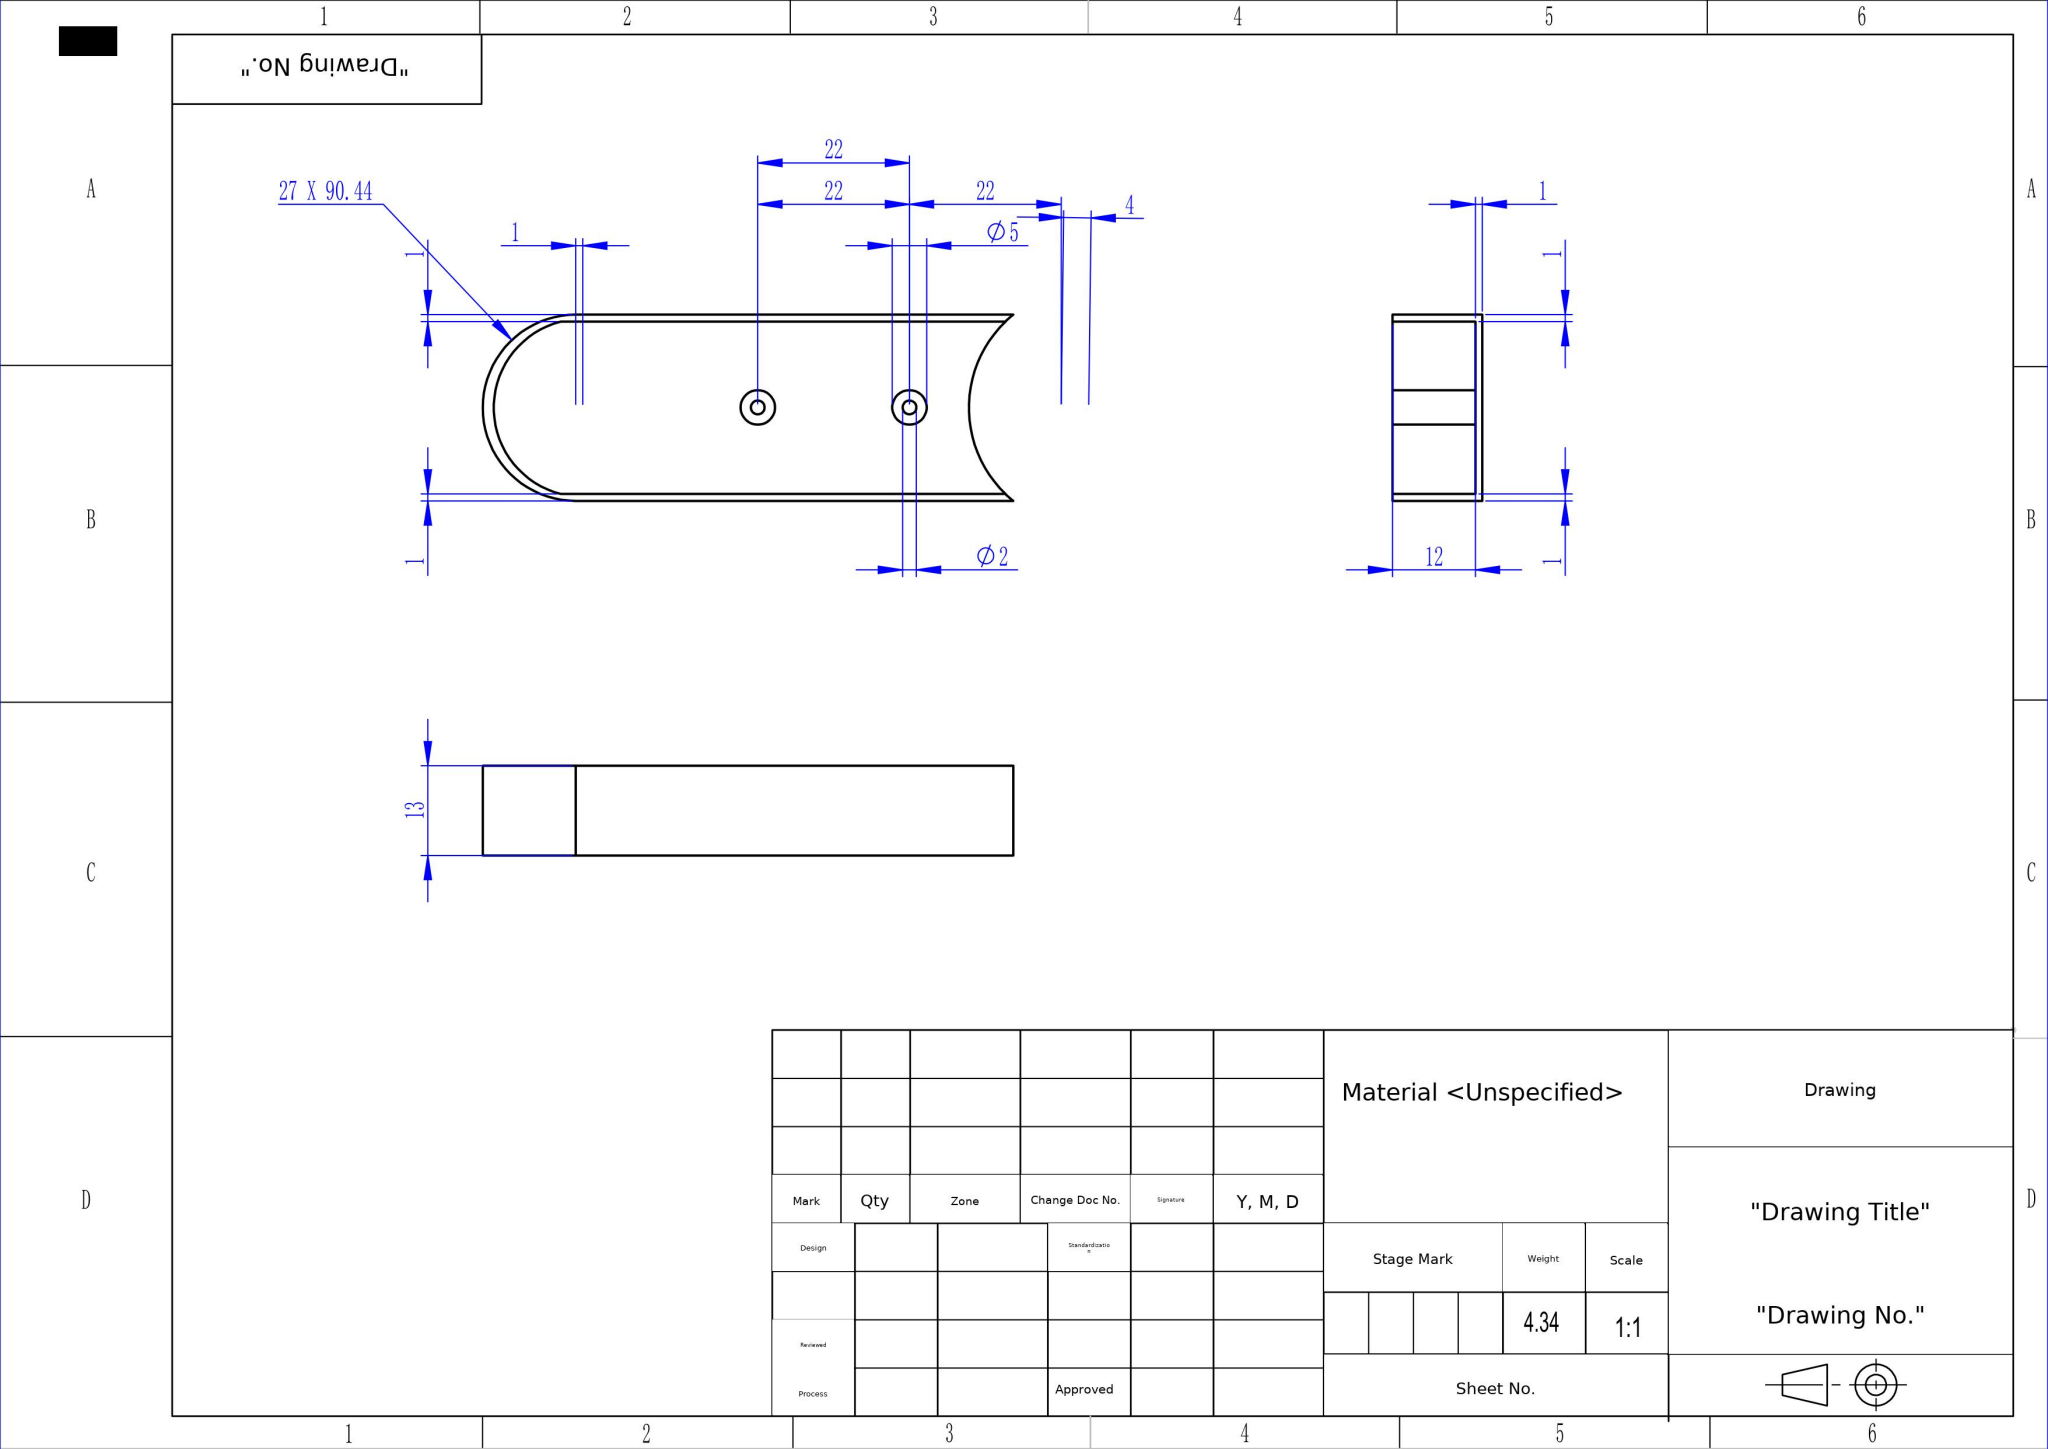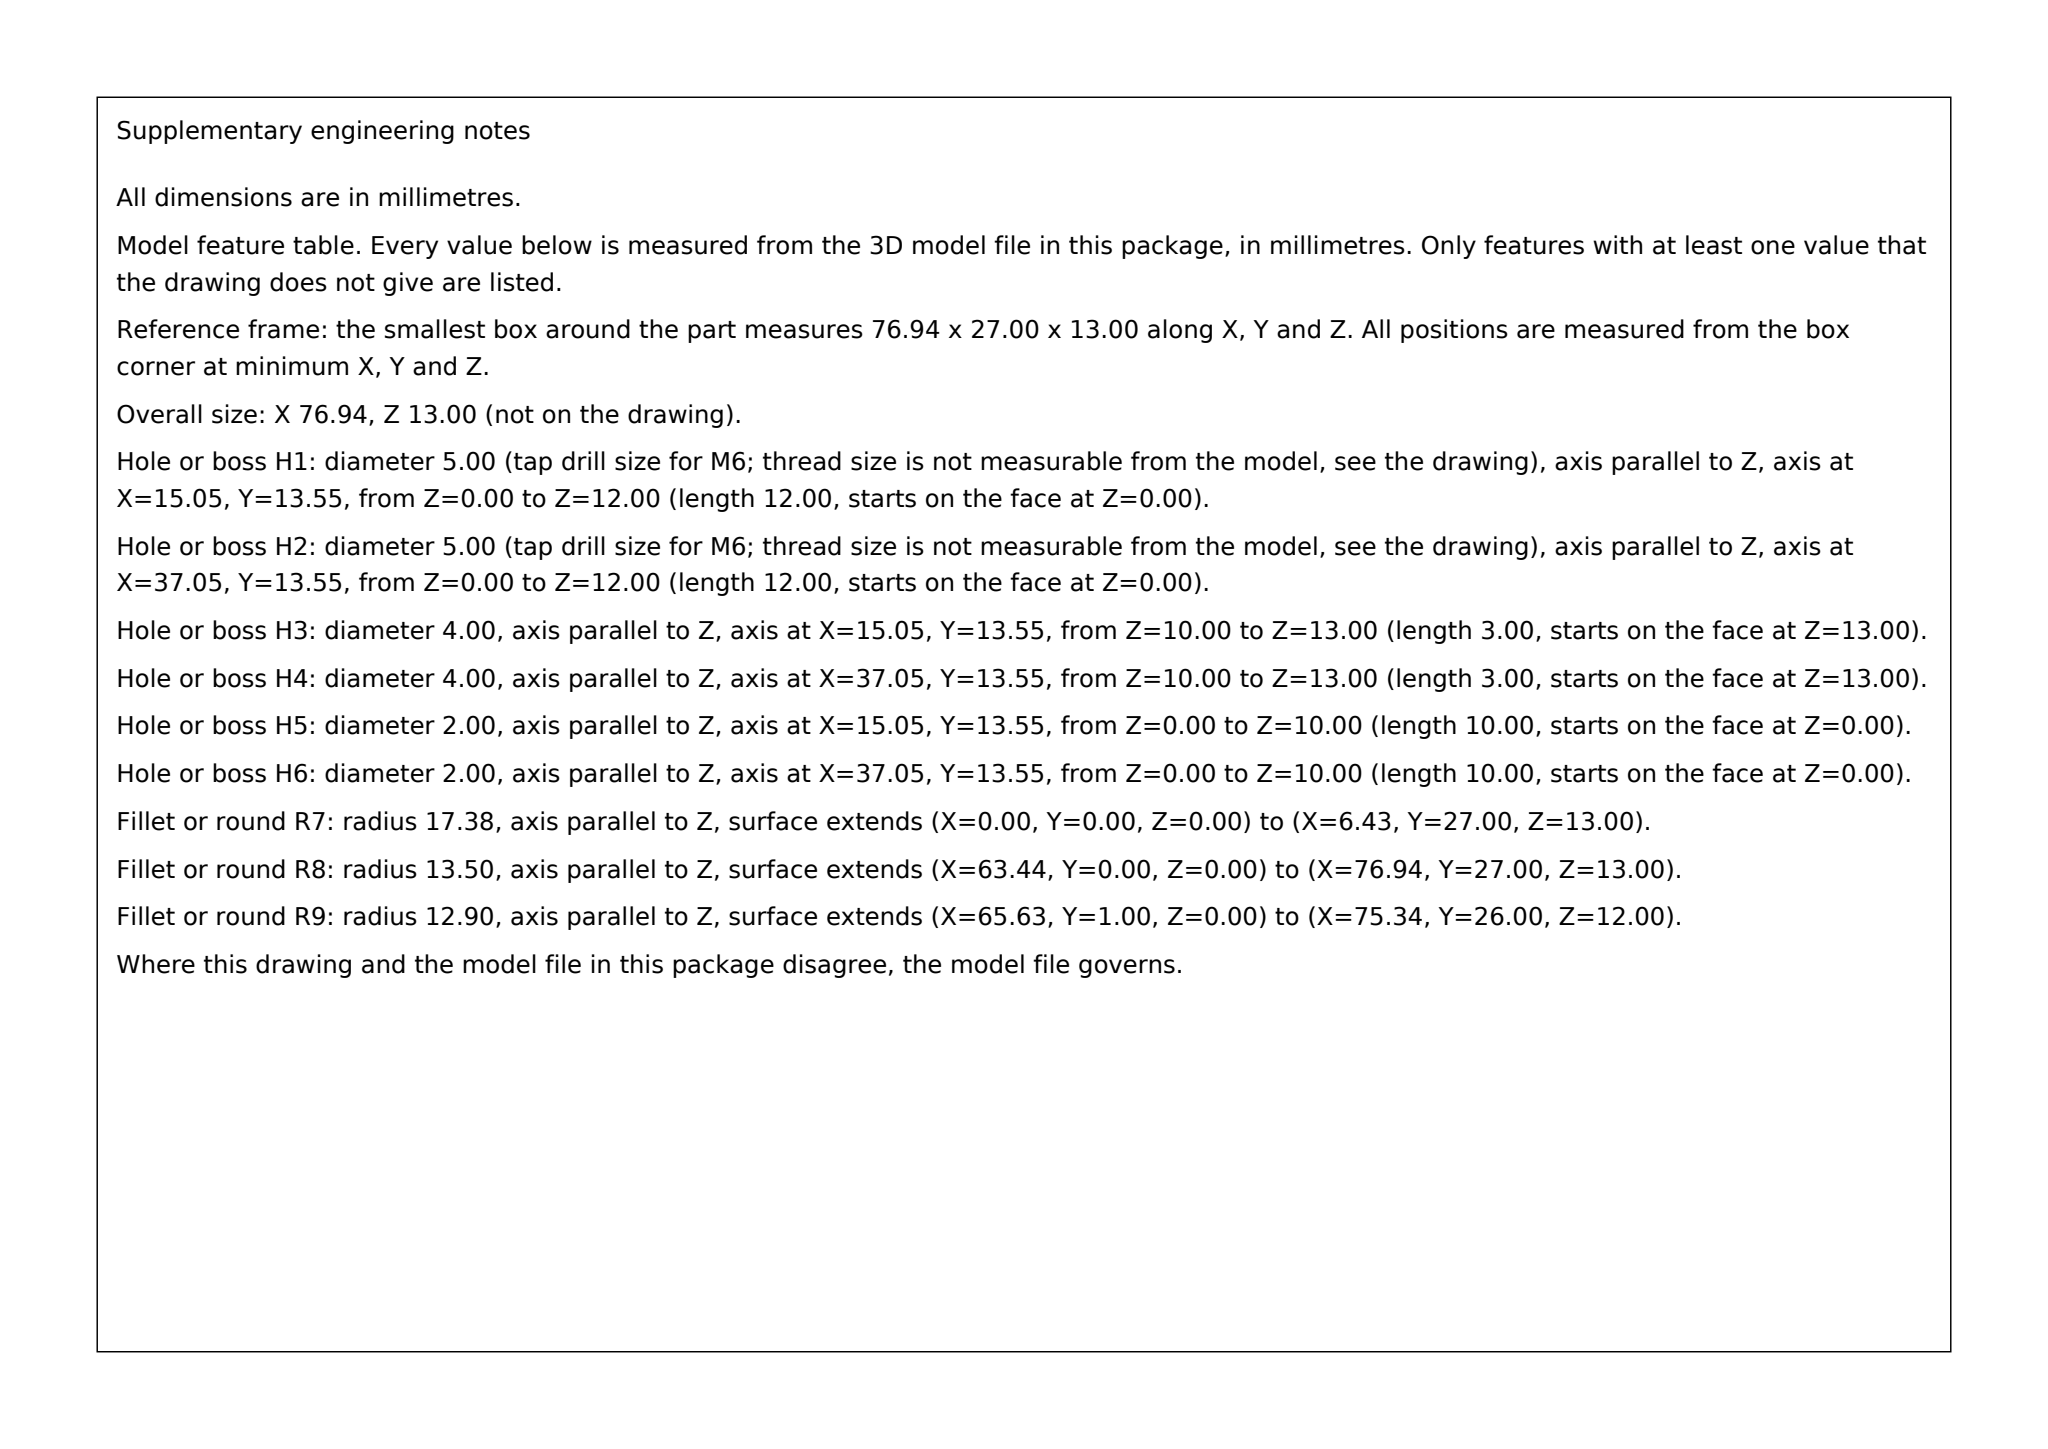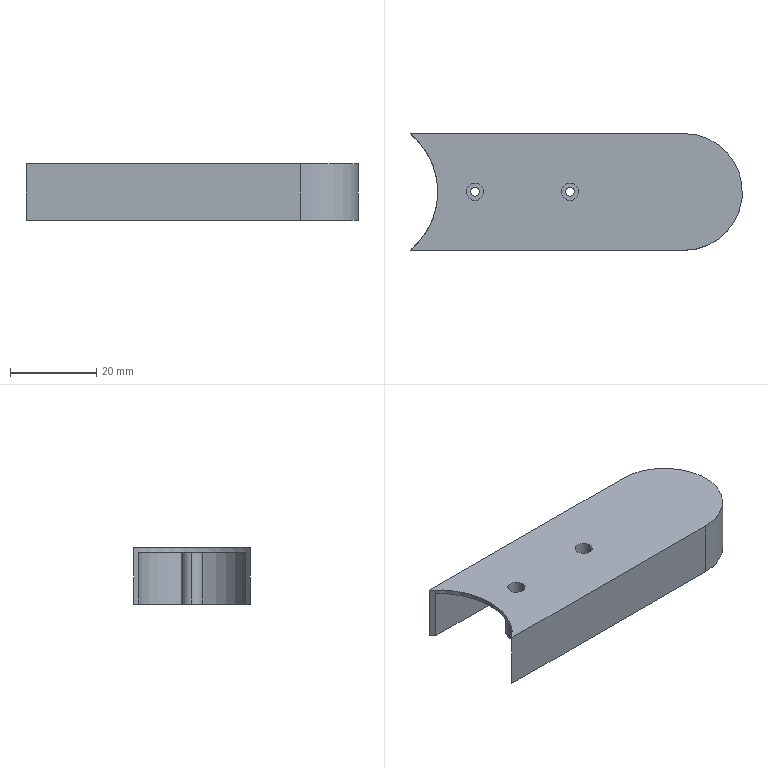Part | SolidWorks | mm | 1 solid | 26 faces | box 76.94 x 27 x 13 mm | volume 4339 mm3 | cylinder 15 | plane 11 | commonest cylinder face diameters 4 x4 5 x4 2 x4 34.768 x1 27 x1 25.801 x1
STEP:
#1=CARTESIAN_POINT('',(-54.,-0.,10.));
#2=VERTEX_POINT('',#1);
#3=CARTESIAN_POINT('',(-50.,-0.,10.));
#4=VERTEX_POINT('',#3);
#5=CARTESIAN_POINT('',(-52.,-0.,10.));
#6=DIRECTION('',(0.,0.,1.));
#7=DIRECTION('',(1.,0.,0.));
#8=AXIS2_PLACEMENT_3D('',#5,#6,#7);
#9=CIRCLE('',#8,2.);
#10=EDGE_CURVE('',#2,#4,#9,.T.);
#11=ORIENTED_EDGE('',*,*,#10,.F.);
#12=CARTESIAN_POINT('',(-54.,-0.,13.));
#13=VERTEX_POINT('',#12);
#14=CARTESIAN_POINT('',(-54.,-0.,10.));
#15=DIRECTION('',(0.,0.,1.));
#16=VECTOR('',#15,1000.);
#17=LINE('',#14,#16);
#18=EDGE_CURVE('',#2,#13,#17,.T.);
#19=ORIENTED_EDGE('',*,*,#18,.T.);
#20=CARTESIAN_POINT('',(-50.,-0.,13.));
#21=VERTEX_POINT('',#20);
#22=CARTESIAN_POINT('',(-52.,-0.,13.));
#23=DIRECTION('',(0.,0.,1.));
#24=DIRECTION('',(1.,0.,0.));
#25=AXIS2_PLACEMENT_3D('',#22,#23,#24);
#26=CIRCLE('',#25,2.);
#27=EDGE_CURVE('',#13,#21,#26,.T.);
#28=ORIENTED_EDGE('',*,*,#27,.T.);
#29=CARTESIAN_POINT('',(-50.,-0.,10.));
#30=DIRECTION('',(0.,0.,1.));
#31=VECTOR('',#30,1000.);
#32=LINE('',#29,#31);
#33=EDGE_CURVE('',#4,#21,#32,.T.);
#34=ORIENTED_EDGE('',*,*,#33,.F.);
#35=EDGE_LOOP('',(#11,#19,#28,#34));
#36=FACE_OUTER_BOUND('',#35,.T.);
#37=CARTESIAN_POINT('',(-52.,-0.,10.));
#38=DIRECTION('',(0.,0.,1.));
#39=DIRECTION('',(1.,0.,0.));
#40=AXIS2_PLACEMENT_3D('',#37,#38,#39);
#41=CYLINDRICAL_SURFACE('',#40,2.);
#42=ADVANCED_FACE('',(#36),#41,.F.);
#43=CARTESIAN_POINT('',(-76.,0.,10.));
#44=VERTEX_POINT('',#43);
#45=CARTESIAN_POINT('',(-72.,0.,10.));
#46=VERTEX_POINT('',#45);
#47=CARTESIAN_POINT('',(-74.,0.,10.));
#48=DIRECTION('',(0.,0.,1.));
#49=DIRECTION('',(1.,0.,0.));
#50=AXIS2_PLACEMENT_3D('',#47,#48,#49);
#51=CIRCLE('',#50,2.);
#52=EDGE_CURVE('',#44,#46,#51,.T.);
#53=ORIENTED_EDGE('',*,*,#52,.F.);
#54=CARTESIAN_POINT('',(-76.,0.,13.));
#55=VERTEX_POINT('',#54);
#56=CARTESIAN_POINT('',(-76.,0.,10.));
#57=DIRECTION('',(0.,0.,1.));
#58=VECTOR('',#57,1000.);
#59=LINE('',#56,#58);
#60=EDGE_CURVE('',#44,#55,#59,.T.);
#61=ORIENTED_EDGE('',*,*,#60,.T.);
#62=CARTESIAN_POINT('',(-72.,0.,13.));
#63=VERTEX_POINT('',#62);
#64=CARTESIAN_POINT('',(-74.,0.,13.));
#65=DIRECTION('',(0.,0.,1.));
#66=DIRECTION('',(1.,0.,0.));
#67=AXIS2_PLACEMENT_3D('',#64,#65,#66);
#68=CIRCLE('',#67,2.);
#69=EDGE_CURVE('',#55,#63,#68,.T.);
#70=ORIENTED_EDGE('',*,*,#69,.T.);
#71=CARTESIAN_POINT('',(-72.,0.,10.));
#72=DIRECTION('',(0.,0.,1.));
#73=VECTOR('',#72,1000.);
#74=LINE('',#71,#73);
#75=EDGE_CURVE('',#46,#63,#74,.T.);
#76=ORIENTED_EDGE('',*,*,#75,.F.);
#77=EDGE_LOOP('',(#53,#61,#70,#76));
#78=FACE_OUTER_BOUND('',#77,.T.);
#79=CARTESIAN_POINT('',(-74.,0.,10.));
#80=DIRECTION('',(0.,0.,1.));
#81=DIRECTION('',(1.,0.,0.));
#82=AXIS2_PLACEMENT_3D('',#79,#80,#81);
#83=CYLINDRICAL_SURFACE('',#82,2.);
#84=ADVANCED_FACE('',(#78),#83,.F.);
#85=CARTESIAN_POINT('',(-54.5,-0.,-0.));
#86=VERTEX_POINT('',#85);
#87=CARTESIAN_POINT('',(-49.5,-0.,-0.));
#88=VERTEX_POINT('',#87);
#89=CARTESIAN_POINT('',(-52.,-0.,-0.));
#90=DIRECTION('',(0.,0.,-1.));
#91=DIRECTION('',(0.,1.,0.));
#92=AXIS2_PLACEMENT_3D('',#89,#90,#91);
#93=CIRCLE('',#92,2.5);
#94=EDGE_CURVE('',#86,#88,#93,.T.);
#95=ORIENTED_EDGE('',*,*,#94,.F.);
#96=CARTESIAN_POINT('',(-54.5,-0.,12.));
#97=VERTEX_POINT('',#96);
#98=CARTESIAN_POINT('',(-54.5,-0.,-7.071));
#99=DIRECTION('',(0.,0.,1.));
#100=VECTOR('',#99,1000.);
#101=LINE('',#98,#100);
#102=EDGE_CURVE('',#86,#97,#101,.T.);
#103=ORIENTED_EDGE('',*,*,#102,.T.);
#104=CARTESIAN_POINT('',(-49.5,-0.,12.));
#105=VERTEX_POINT('',#104);
#106=CARTESIAN_POINT('',(-52.,-0.,12.));
#107=DIRECTION('',(0.,0.,-1.));
#108=DIRECTION('',(-1.,0.,0.));
#109=AXIS2_PLACEMENT_3D('',#106,#107,#108);
#110=CIRCLE('',#109,2.5);
#111=EDGE_CURVE('',#97,#105,#110,.T.);
#112=ORIENTED_EDGE('',*,*,#111,.T.);
#113=CARTESIAN_POINT('',(-49.5,-0.,-7.071));
#114=DIRECTION('',(0.,0.,1.));
#115=VECTOR('',#114,1000.);
#116=LINE('',#113,#115);
#117=EDGE_CURVE('',#88,#105,#116,.T.);
#118=ORIENTED_EDGE('',*,*,#117,.F.);
#119=EDGE_LOOP('',(#95,#103,#112,#118));
#120=FACE_OUTER_BOUND('',#119,.T.);
#121=CARTESIAN_POINT('',(-52.,-0.,-7.071));
#122=DIRECTION('',(0.,0.,1.));
#123=DIRECTION('',(1.,0.,0.));
#124=AXIS2_PLACEMENT_3D('',#121,#122,#123);
#125=CYLINDRICAL_SURFACE('',#124,2.5);
#126=ADVANCED_FACE('',(#120),#125,.T.);
#127=CARTESIAN_POINT('',(-76.5,0.,-0.));
#128=VERTEX_POINT('',#127);
#129=CARTESIAN_POINT('',(-71.5,0.,-0.));
#130=VERTEX_POINT('',#129);
#131=CARTESIAN_POINT('',(-74.,0.,-0.));
#132=DIRECTION('',(0.,0.,-1.));
#133=DIRECTION('',(0.,1.,0.));
#134=AXIS2_PLACEMENT_3D('',#131,#132,#133);
#135=CIRCLE('',#134,2.5);
#136=EDGE_CURVE('',#128,#130,#135,.T.);
#137=ORIENTED_EDGE('',*,*,#136,.F.);
#138=CARTESIAN_POINT('',(-76.5,0.,12.));
#139=VERTEX_POINT('',#138);
#140=CARTESIAN_POINT('',(-76.5,0.,-7.071));
#141=DIRECTION('',(0.,0.,1.));
#142=VECTOR('',#141,1000.);
#143=LINE('',#140,#142);
#144=EDGE_CURVE('',#128,#139,#143,.T.);
#145=ORIENTED_EDGE('',*,*,#144,.T.);
#146=CARTESIAN_POINT('',(-71.5,0.,12.));
#147=VERTEX_POINT('',#146);
#148=CARTESIAN_POINT('',(-74.,0.,12.));
#149=DIRECTION('',(0.,0.,-1.));
#150=DIRECTION('',(-1.,0.,0.));
#151=AXIS2_PLACEMENT_3D('',#148,#149,#150);
#152=CIRCLE('',#151,2.5);
#153=EDGE_CURVE('',#139,#147,#152,.T.);
#154=ORIENTED_EDGE('',*,*,#153,.T.);
#155=CARTESIAN_POINT('',(-71.5,0.,-7.071));
#156=DIRECTION('',(0.,0.,1.));
#157=VECTOR('',#156,1000.);
#158=LINE('',#155,#157);
#159=EDGE_CURVE('',#130,#147,#158,.T.);
#160=ORIENTED_EDGE('',*,*,#159,.F.);
#161=EDGE_LOOP('',(#137,#145,#154,#160));
#162=FACE_OUTER_BOUND('',#161,.T.);
#163=CARTESIAN_POINT('',(-74.,0.,-7.071));
#164=DIRECTION('',(0.,0.,1.));
#165=DIRECTION('',(1.,0.,0.));
#166=AXIS2_PLACEMENT_3D('',#163,#164,#165);
#167=CYLINDRICAL_SURFACE('',#166,2.5);
#168=ADVANCED_FACE('',(#162),#167,.T.);
#169=CARTESIAN_POINT('',(-75.,0.,-0.));
#170=VERTEX_POINT('',#169);
#171=CARTESIAN_POINT('',(-73.,0.,-0.));
#172=VERTEX_POINT('',#171);
#173=CARTESIAN_POINT('',(-74.,0.,-0.));
#174=DIRECTION('',(0.,0.,1.));
#175=DIRECTION('',(1.,0.,0.));
#176=AXIS2_PLACEMENT_3D('',#173,#174,#175);
#177=CIRCLE('',#176,1.);
#178=EDGE_CURVE('',#170,#172,#177,.T.);
#179=ORIENTED_EDGE('',*,*,#178,.F.);
#180=CARTESIAN_POINT('',(-75.,0.,10.));
#181=VERTEX_POINT('',#180);
#182=CARTESIAN_POINT('',(-75.,0.,-0.));
#183=DIRECTION('',(0.,0.,1.));
#184=VECTOR('',#183,1000.);
#185=LINE('',#182,#184);
#186=EDGE_CURVE('',#170,#181,#185,.T.);
#187=ORIENTED_EDGE('',*,*,#186,.T.);
#188=CARTESIAN_POINT('',(-73.,0.,10.));
#189=VERTEX_POINT('',#188);
#190=CARTESIAN_POINT('',(-74.,0.,10.));
#191=DIRECTION('',(0.,0.,-1.));
#192=DIRECTION('',(1.,0.,0.));
#193=AXIS2_PLACEMENT_3D('',#190,#191,#192);
#194=CIRCLE('',#193,1.);
#195=EDGE_CURVE('',#189,#181,#194,.T.);
#196=ORIENTED_EDGE('',*,*,#195,.F.);
#197=CARTESIAN_POINT('',(-73.,0.,-0.));
#198=DIRECTION('',(0.,0.,1.));
#199=VECTOR('',#198,1000.);
#200=LINE('',#197,#199);
#201=EDGE_CURVE('',#172,#189,#200,.T.);
#202=ORIENTED_EDGE('',*,*,#201,.F.);
#203=EDGE_LOOP('',(#179,#187,#196,#202));
#204=FACE_OUTER_BOUND('',#203,.T.);
#205=CARTESIAN_POINT('',(-74.,0.,-0.));
#206=DIRECTION('',(0.,0.,1.));
#207=DIRECTION('',(1.,0.,0.));
#208=AXIS2_PLACEMENT_3D('',#205,#206,#207);
#209=CYLINDRICAL_SURFACE('',#208,1.);
#210=ADVANCED_FACE('',(#204),#209,.F.);
#211=CARTESIAN_POINT('',(-53.,-0.,-0.));
#212=VERTEX_POINT('',#211);
#213=CARTESIAN_POINT('',(-51.,-0.,-0.));
#214=VERTEX_POINT('',#213);
#215=CARTESIAN_POINT('',(-52.,-0.,-0.));
#216=DIRECTION('',(0.,0.,1.));
#217=DIRECTION('',(1.,0.,0.));
#218=AXIS2_PLACEMENT_3D('',#215,#216,#217);
#219=CIRCLE('',#218,1.);
#220=EDGE_CURVE('',#212,#214,#219,.T.);
#221=ORIENTED_EDGE('',*,*,#220,.F.);
#222=CARTESIAN_POINT('',(-53.,-0.,10.));
#223=VERTEX_POINT('',#222);
#224=CARTESIAN_POINT('',(-53.,-0.,-0.));
#225=DIRECTION('',(0.,0.,1.));
#226=VECTOR('',#225,1000.);
#227=LINE('',#224,#226);
#228=EDGE_CURVE('',#212,#223,#227,.T.);
#229=ORIENTED_EDGE('',*,*,#228,.T.);
#230=CARTESIAN_POINT('',(-51.,-0.,10.));
#231=VERTEX_POINT('',#230);
#232=CARTESIAN_POINT('',(-52.,-0.,10.));
#233=DIRECTION('',(0.,0.,-1.));
#234=DIRECTION('',(1.,0.,0.));
#235=AXIS2_PLACEMENT_3D('',#232,#233,#234);
#236=CIRCLE('',#235,1.);
#237=EDGE_CURVE('',#231,#223,#236,.T.);
#238=ORIENTED_EDGE('',*,*,#237,.F.);
#239=CARTESIAN_POINT('',(-51.,-0.,-0.));
#240=DIRECTION('',(0.,0.,1.));
#241=VECTOR('',#240,1000.);
#242=LINE('',#239,#241);
#243=EDGE_CURVE('',#214,#231,#242,.T.);
#244=ORIENTED_EDGE('',*,*,#243,.F.);
#245=EDGE_LOOP('',(#221,#229,#238,#244));
#246=FACE_OUTER_BOUND('',#245,.T.);
#247=CARTESIAN_POINT('',(-52.,-0.,-0.));
#248=DIRECTION('',(0.,0.,1.));
#249=DIRECTION('',(1.,0.,0.));
#250=AXIS2_PLACEMENT_3D('',#247,#248,#249);
#251=CYLINDRICAL_SURFACE('',#250,1.);
#252=ADVANCED_FACE('',(#246),#251,.F.);
#253=ORIENTED_EDGE('',*,*,#228,.F.);
#254=CARTESIAN_POINT('',(-52.,-0.,-0.));
#255=DIRECTION('',(0.,0.,1.));
#256=DIRECTION('',(1.,0.,0.));
#257=AXIS2_PLACEMENT_3D('',#254,#255,#256);
#258=CIRCLE('',#257,1.);
#259=EDGE_CURVE('',#214,#212,#258,.T.);
#260=ORIENTED_EDGE('',*,*,#259,.F.);
#261=ORIENTED_EDGE('',*,*,#243,.T.);
#262=CARTESIAN_POINT('',(-52.,-0.,10.));
#263=DIRECTION('',(0.,0.,-1.));
#264=DIRECTION('',(1.,0.,0.));
#265=AXIS2_PLACEMENT_3D('',#262,#263,#264);
#266=CIRCLE('',#265,1.);
#267=EDGE_CURVE('',#223,#231,#266,.T.);
#268=ORIENTED_EDGE('',*,*,#267,.F.);
#269=EDGE_LOOP('',(#253,#260,#261,#268));
#270=FACE_OUTER_BOUND('',#269,.T.);
#271=CARTESIAN_POINT('',(-52.,-0.,-0.));
#272=DIRECTION('',(0.,0.,1.));
#273=DIRECTION('',(1.,0.,0.));
#274=AXIS2_PLACEMENT_3D('',#271,#272,#273);
#275=CYLINDRICAL_SURFACE('',#274,1.);
#276=ADVANCED_FACE('',(#270),#275,.F.);
#277=ORIENTED_EDGE('',*,*,#186,.F.);
#278=CARTESIAN_POINT('',(-74.,0.,-0.));
#279=DIRECTION('',(0.,0.,1.));
#280=DIRECTION('',(1.,0.,0.));
#281=AXIS2_PLACEMENT_3D('',#278,#279,#280);
#282=CIRCLE('',#281,1.);
#283=EDGE_CURVE('',#172,#170,#282,.T.);
#284=ORIENTED_EDGE('',*,*,#283,.F.);
#285=ORIENTED_EDGE('',*,*,#201,.T.);
#286=CARTESIAN_POINT('',(-74.,0.,10.));
#287=DIRECTION('',(0.,0.,-1.));
#288=DIRECTION('',(1.,0.,0.));
#289=AXIS2_PLACEMENT_3D('',#286,#287,#288);
#290=CIRCLE('',#289,1.);
#291=EDGE_CURVE('',#181,#189,#290,.T.);
#292=ORIENTED_EDGE('',*,*,#291,.F.);
#293=EDGE_LOOP('',(#277,#284,#285,#292));
#294=FACE_OUTER_BOUND('',#293,.T.);
#295=CARTESIAN_POINT('',(-74.,0.,-0.));
#296=DIRECTION('',(0.,0.,1.));
#297=DIRECTION('',(1.,0.,0.));
#298=AXIS2_PLACEMENT_3D('',#295,#296,#297);
#299=CYLINDRICAL_SURFACE('',#298,1.);
#300=ADVANCED_FACE('',(#294),#299,.F.);
#301=CARTESIAN_POINT('',(-89.048,13.45,0.));
#302=VERTEX_POINT('',#301);
#303=CARTESIAN_POINT('',(-87.919,12.45,0.));
#304=VERTEX_POINT('',#303);
#305=CARTESIAN_POINT('',(-100.,-0.05,0.));
#306=DIRECTION('',(0.,0.,-1.));
#307=DIRECTION('',(1.,-0.,0.));
#308=AXIS2_PLACEMENT_3D('',#305,#306,#307);
#309=CIRCLE('',#308,17.384);
#310=EDGE_CURVE('',#302,#304,#309,.T.);
#311=ORIENTED_EDGE('',*,*,#310,.T.);
#312=CARTESIAN_POINT('',(-87.919,12.45,12.));
#313=VERTEX_POINT('',#312);
#314=CARTESIAN_POINT('',(-87.919,12.45,12.));
#315=DIRECTION('',(0.,0.,-1.));
#316=VECTOR('',#315,1000.);
#317=LINE('',#314,#316);
#318=EDGE_CURVE('',#313,#304,#317,.T.);
#319=ORIENTED_EDGE('',*,*,#318,.F.);
#320=CARTESIAN_POINT('',(-87.919,-12.55,12.));
#321=VERTEX_POINT('',#320);
#322=CARTESIAN_POINT('',(-100.,-0.05,12.));
#323=DIRECTION('',(0.,0.,1.));
#324=DIRECTION('',(-1.,0.,0.));
#325=AXIS2_PLACEMENT_3D('',#322,#323,#324);
#326=CIRCLE('',#325,17.384);
#327=EDGE_CURVE('',#321,#313,#326,.T.);
#328=ORIENTED_EDGE('',*,*,#327,.F.);
#329=CARTESIAN_POINT('',(-87.919,-12.55,0.));
#330=VERTEX_POINT('',#329);
#331=CARTESIAN_POINT('',(-87.919,-12.55,12.));
#332=DIRECTION('',(0.,0.,-1.));
#333=VECTOR('',#332,1000.);
#334=LINE('',#331,#333);
#335=EDGE_CURVE('',#321,#330,#334,.T.);
#336=ORIENTED_EDGE('',*,*,#335,.T.);
#337=CARTESIAN_POINT('',(-89.048,-13.55,0.));
#338=VERTEX_POINT('',#337);
#339=CARTESIAN_POINT('',(-100.,-0.05,0.));
#340=DIRECTION('',(0.,0.,-1.));
#341=DIRECTION('',(1.,0.,0.));
#342=AXIS2_PLACEMENT_3D('',#339,#340,#341);
#343=CIRCLE('',#342,17.384);
#344=EDGE_CURVE('',#330,#338,#343,.T.);
#345=ORIENTED_EDGE('',*,*,#344,.T.);
#346=CARTESIAN_POINT('',(-89.048,-13.55,13.));
#347=VERTEX_POINT('',#346);
#348=CARTESIAN_POINT('',(-89.048,-13.55,13.));
#349=DIRECTION('',(0.,0.,-1.));
#350=VECTOR('',#349,1000.);
#351=LINE('',#348,#350);
#352=EDGE_CURVE('',#347,#338,#351,.T.);
#353=ORIENTED_EDGE('',*,*,#352,.F.);
#354=CARTESIAN_POINT('',(-89.048,13.45,13.));
#355=VERTEX_POINT('',#354);
#356=CARTESIAN_POINT('',(-100.,-0.05,13.));
#357=DIRECTION('',(0.,0.,-1.));
#358=DIRECTION('',(1.,0.,0.));
#359=AXIS2_PLACEMENT_3D('',#356,#357,#358);
#360=CIRCLE('',#359,17.384);
#361=EDGE_CURVE('',#355,#347,#360,.T.);
#362=ORIENTED_EDGE('',*,*,#361,.F.);
#363=CARTESIAN_POINT('',(-89.048,13.45,13.));
#364=DIRECTION('',(0.,0.,-1.));
#365=VECTOR('',#364,1000.);
#366=LINE('',#363,#365);
#367=EDGE_CURVE('',#355,#302,#366,.T.);
#368=ORIENTED_EDGE('',*,*,#367,.T.);
#369=EDGE_LOOP('',(#311,#319,#328,#336,#345,#353,#362,#368));
#370=FACE_OUTER_BOUND('',#369,.T.);
#371=CARTESIAN_POINT('',(-100.,-0.05,13.));
#372=DIRECTION('',(0.,0.,-1.));
#373=DIRECTION('',(-1.,0.,0.));
#374=AXIS2_PLACEMENT_3D('',#371,#372,#373);
#375=CYLINDRICAL_SURFACE('',#374,17.384);
#376=ADVANCED_FACE('',(#370),#375,.F.);
#377=CARTESIAN_POINT('',(-25.611,-13.55,0.));
#378=VERTEX_POINT('',#377);
#379=CARTESIAN_POINT('',(0.,-13.55,0.));
#380=DIRECTION('',(-1.,0.,0.));
#381=VECTOR('',#380,1000.);
#382=LINE('',#379,#381);
#383=EDGE_CURVE('',#378,#338,#382,.T.);
#384=ORIENTED_EDGE('',*,*,#383,.F.);
#385=CARTESIAN_POINT('',(-25.611,-13.55,13.));
#386=VERTEX_POINT('',#385);
#387=CARTESIAN_POINT('',(-25.611,-13.55,13.));
#388=DIRECTION('',(0.,0.,-1.));
#389=VECTOR('',#388,1000.);
#390=LINE('',#387,#389);
#391=EDGE_CURVE('',#386,#378,#390,.T.);
#392=ORIENTED_EDGE('',*,*,#391,.F.);
#393=CARTESIAN_POINT('',(0.,-13.55,13.));
#394=DIRECTION('',(-1.,0.,0.));
#395=VECTOR('',#394,1000.);
#396=LINE('',#393,#395);
#397=EDGE_CURVE('',#386,#347,#396,.T.);
#398=ORIENTED_EDGE('',*,*,#397,.T.);
#399=ORIENTED_EDGE('',*,*,#352,.T.);
#400=EDGE_LOOP('',(#384,#392,#398,#399));
#401=FACE_OUTER_BOUND('',#400,.T.);
#402=CARTESIAN_POINT('',(0.,-13.55,13.));
#403=DIRECTION('',(0.,-1.,0.));
#404=DIRECTION('',(0.,0.,-1.));
#405=AXIS2_PLACEMENT_3D('',#402,#403,#404);
#406=PLANE('',#405);
#407=ADVANCED_FACE('',(#401),#406,.T.);
#408=CARTESIAN_POINT('',(-25.611,13.45,0.));
#409=VERTEX_POINT('',#408);
#410=CARTESIAN_POINT('',(-25.611,-0.05,0.));
#411=DIRECTION('',(0.,0.,1.));
#412=DIRECTION('',(1.,0.,0.));
#413=AXIS2_PLACEMENT_3D('',#410,#411,#412);
#414=CIRCLE('',#413,13.5);
#415=EDGE_CURVE('',#378,#409,#414,.T.);
#416=ORIENTED_EDGE('',*,*,#415,.T.);
#417=CARTESIAN_POINT('',(-25.611,13.45,13.));
#418=VERTEX_POINT('',#417);
#419=CARTESIAN_POINT('',(-25.611,13.45,13.));
#420=DIRECTION('',(0.,0.,-1.));
#421=VECTOR('',#420,1000.);
#422=LINE('',#419,#421);
#423=EDGE_CURVE('',#418,#409,#422,.T.);
#424=ORIENTED_EDGE('',*,*,#423,.F.);
#425=CARTESIAN_POINT('',(-25.611,-0.05,13.));
#426=DIRECTION('',(0.,0.,1.));
#427=DIRECTION('',(1.,0.,0.));
#428=AXIS2_PLACEMENT_3D('',#425,#426,#427);
#429=CIRCLE('',#428,13.5);
#430=EDGE_CURVE('',#386,#418,#429,.T.);
#431=ORIENTED_EDGE('',*,*,#430,.F.);
#432=ORIENTED_EDGE('',*,*,#391,.T.);
#433=EDGE_LOOP('',(#416,#424,#431,#432));
#434=FACE_OUTER_BOUND('',#433,.T.);
#435=CARTESIAN_POINT('',(-25.611,-0.05,13.));
#436=DIRECTION('',(0.,0.,-1.));
#437=DIRECTION('',(-1.,0.,0.));
#438=AXIS2_PLACEMENT_3D('',#435,#436,#437);
#439=CYLINDRICAL_SURFACE('',#438,13.5);
#440=ADVANCED_FACE('',(#434),#439,.T.);
#441=CARTESIAN_POINT('',(0.,13.45,0.));
#442=DIRECTION('',(-1.,0.,0.));
#443=VECTOR('',#442,1000.);
#444=LINE('',#441,#443);
#445=EDGE_CURVE('',#409,#302,#444,.T.);
#446=ORIENTED_EDGE('',*,*,#445,.T.);
#447=ORIENTED_EDGE('',*,*,#367,.F.);
#448=CARTESIAN_POINT('',(0.,13.45,13.));
#449=DIRECTION('',(-1.,0.,0.));
#450=VECTOR('',#449,1000.);
#451=LINE('',#448,#450);
#452=EDGE_CURVE('',#418,#355,#451,.T.);
#453=ORIENTED_EDGE('',*,*,#452,.F.);
#454=ORIENTED_EDGE('',*,*,#423,.T.);
#455=EDGE_LOOP('',(#446,#447,#453,#454));
#456=FACE_OUTER_BOUND('',#455,.T.);
#457=CARTESIAN_POINT('',(0.,13.45,13.));
#458=DIRECTION('',(0.,-1.,0.));
#459=DIRECTION('',(0.,0.,-1.));
#460=AXIS2_PLACEMENT_3D('',#457,#458,#459);
#461=PLANE('',#460);
#462=ADVANCED_FACE('',(#456),#461,.F.);
#463=CARTESIAN_POINT('',(-74.,0.,13.));
#464=DIRECTION('',(0.,0.,1.));
#465=DIRECTION('',(1.,0.,0.));
#466=AXIS2_PLACEMENT_3D('',#463,#464,#465);
#467=CIRCLE('',#466,2.);
#468=EDGE_CURVE('',#63,#55,#467,.T.);
#469=ORIENTED_EDGE('',*,*,#468,.F.);
#470=ORIENTED_EDGE('',*,*,#69,.F.);
#471=EDGE_LOOP('',(#469,#470));
#472=FACE_BOUND('',#471,.T.);
#473=CARTESIAN_POINT('',(-52.,-0.,13.));
#474=DIRECTION('',(0.,0.,1.));
#475=DIRECTION('',(1.,0.,0.));
#476=AXIS2_PLACEMENT_3D('',#473,#474,#475);
#477=CIRCLE('',#476,2.);
#478=EDGE_CURVE('',#21,#13,#477,.T.);
#479=ORIENTED_EDGE('',*,*,#478,.F.);
#480=ORIENTED_EDGE('',*,*,#27,.F.);
#481=EDGE_LOOP('',(#479,#480));
#482=FACE_BOUND('',#481,.T.);
#483=ORIENTED_EDGE('',*,*,#361,.T.);
#484=ORIENTED_EDGE('',*,*,#397,.F.);
#485=ORIENTED_EDGE('',*,*,#430,.T.);
#486=ORIENTED_EDGE('',*,*,#452,.T.);
#487=EDGE_LOOP('',(#483,#484,#485,#486));
#488=FACE_OUTER_BOUND('',#487,.T.);
#489=CARTESIAN_POINT('',(0.,0.,13.));
#490=DIRECTION('',(0.,0.,1.));
#491=DIRECTION('',(1.,0.,0.));
#492=AXIS2_PLACEMENT_3D('',#489,#490,#491);
#493=PLANE('',#492);
#494=ADVANCED_FACE('',(#472,#482,#488),#493,.T.);
#495=CARTESIAN_POINT('',(-23.421,12.45,0.));
#496=VERTEX_POINT('',#495);
#497=CARTESIAN_POINT('',(-23.421,-12.55,0.));
#498=VERTEX_POINT('',#497);
#499=CARTESIAN_POINT('',(-26.611,-0.05,0.));
#500=DIRECTION('',(0.,0.,-1.));
#501=DIRECTION('',(-1.,0.,0.));
#502=AXIS2_PLACEMENT_3D('',#499,#500,#501);
#503=CIRCLE('',#502,12.9);
#504=EDGE_CURVE('',#496,#498,#503,.T.);
#505=ORIENTED_EDGE('',*,*,#504,.F.);
#506=CARTESIAN_POINT('',(0.,12.45,0.));
#507=DIRECTION('',(1.,-0.,0.));
#508=VECTOR('',#507,1000.);
#509=LINE('',#506,#508);
#510=EDGE_CURVE('',#304,#496,#509,.T.);
#511=ORIENTED_EDGE('',*,*,#510,.F.);
#512=ORIENTED_EDGE('',*,*,#310,.F.);
#513=ORIENTED_EDGE('',*,*,#445,.F.);
#514=ORIENTED_EDGE('',*,*,#415,.F.);
#515=ORIENTED_EDGE('',*,*,#383,.T.);
#516=ORIENTED_EDGE('',*,*,#344,.F.);
#517=CARTESIAN_POINT('',(-0.,-12.55,0.));
#518=DIRECTION('',(-1.,0.,0.));
#519=VECTOR('',#518,1000.);
#520=LINE('',#517,#519);
#521=EDGE_CURVE('',#498,#330,#520,.T.);
#522=ORIENTED_EDGE('',*,*,#521,.F.);
#523=EDGE_LOOP('',(#505,#511,#512,#513,#514,#515,#516,#522));
#524=FACE_OUTER_BOUND('',#523,.T.);
#525=CARTESIAN_POINT('',(0.,0.,0.));
#526=DIRECTION('',(0.,0.,1.));
#527=DIRECTION('',(1.,0.,0.));
#528=AXIS2_PLACEMENT_3D('',#525,#526,#527);
#529=PLANE('',#528);
#530=ADVANCED_FACE('',(#524),#529,.F.);
#531=ORIENTED_EDGE('',*,*,#510,.T.);
#532=CARTESIAN_POINT('',(-23.421,12.45,12.));
#533=VERTEX_POINT('',#532);
#534=CARTESIAN_POINT('',(-23.421,12.45,12.));
#535=DIRECTION('',(0.,0.,-1.));
#536=VECTOR('',#535,1000.);
#537=LINE('',#534,#536);
#538=EDGE_CURVE('',#533,#496,#537,.T.);
#539=ORIENTED_EDGE('',*,*,#538,.F.);
#540=CARTESIAN_POINT('',(0.,12.45,12.));
#541=DIRECTION('',(1.,-0.,0.));
#542=VECTOR('',#541,1000.);
#543=LINE('',#540,#542);
#544=EDGE_CURVE('',#313,#533,#543,.T.);
#545=ORIENTED_EDGE('',*,*,#544,.F.);
#546=ORIENTED_EDGE('',*,*,#318,.T.);
#547=EDGE_LOOP('',(#531,#539,#545,#546));
#548=FACE_OUTER_BOUND('',#547,.T.);
#549=CARTESIAN_POINT('',(0.,12.45,12.));
#550=DIRECTION('',(0.,1.,0.));
#551=DIRECTION('',(-1.,0.,0.));
#552=AXIS2_PLACEMENT_3D('',#549,#550,#551);
#553=PLANE('',#552);
#554=ADVANCED_FACE('',(#548),#553,.F.);
#555=ORIENTED_EDGE('',*,*,#521,.T.);
#556=ORIENTED_EDGE('',*,*,#335,.F.);
#557=CARTESIAN_POINT('',(-23.421,-12.55,12.));
#558=VERTEX_POINT('',#557);
#559=CARTESIAN_POINT('',(-0.,-12.55,12.));
#560=DIRECTION('',(-1.,0.,0.));
#561=VECTOR('',#560,1000.);
#562=LINE('',#559,#561);
#563=EDGE_CURVE('',#558,#321,#562,.T.);
#564=ORIENTED_EDGE('',*,*,#563,.F.);
#565=CARTESIAN_POINT('',(-23.421,-12.55,12.));
#566=DIRECTION('',(0.,0.,-1.));
#567=VECTOR('',#566,1000.);
#568=LINE('',#565,#567);
#569=EDGE_CURVE('',#558,#498,#568,.T.);
#570=ORIENTED_EDGE('',*,*,#569,.T.);
#571=EDGE_LOOP('',(#555,#556,#564,#570));
#572=FACE_OUTER_BOUND('',#571,.T.);
#573=CARTESIAN_POINT('',(-0.,-12.55,12.));
#574=DIRECTION('',(-0.,-1.,0.));
#575=DIRECTION('',(1.,-0.,0.));
#576=AXIS2_PLACEMENT_3D('',#573,#574,#575);
#577=PLANE('',#576);
#578=ADVANCED_FACE('',(#572),#577,.F.);
#579=ORIENTED_EDGE('',*,*,#504,.T.);
#580=ORIENTED_EDGE('',*,*,#569,.F.);
#581=CARTESIAN_POINT('',(-26.611,-0.05,12.));
#582=DIRECTION('',(0.,0.,-1.));
#583=DIRECTION('',(-1.,0.,0.));
#584=AXIS2_PLACEMENT_3D('',#581,#582,#583);
#585=CIRCLE('',#584,12.9);
#586=EDGE_CURVE('',#533,#558,#585,.T.);
#587=ORIENTED_EDGE('',*,*,#586,.F.);
#588=ORIENTED_EDGE('',*,*,#538,.T.);
#589=EDGE_LOOP('',(#579,#580,#587,#588));
#590=FACE_OUTER_BOUND('',#589,.T.);
#591=CARTESIAN_POINT('',(-26.611,-0.05,12.));
#592=DIRECTION('',(0.,0.,-1.));
#593=DIRECTION('',(-1.,0.,0.));
#594=AXIS2_PLACEMENT_3D('',#591,#592,#593);
#595=CYLINDRICAL_SURFACE('',#594,12.9);
#596=ADVANCED_FACE('',(#590),#595,.F.);
#597=CARTESIAN_POINT('',(-52.,-0.,12.));
#598=DIRECTION('',(0.,0.,-1.));
#599=DIRECTION('',(-1.,0.,0.));
#600=AXIS2_PLACEMENT_3D('',#597,#598,#599);
#601=CIRCLE('',#600,2.5);
#602=EDGE_CURVE('',#105,#97,#601,.T.);
#603=ORIENTED_EDGE('',*,*,#602,.F.);
#604=ORIENTED_EDGE('',*,*,#111,.F.);
#605=EDGE_LOOP('',(#603,#604));
#606=FACE_BOUND('',#605,.T.);
#607=CARTESIAN_POINT('',(-74.,0.,12.));
#608=DIRECTION('',(0.,0.,-1.));
#609=DIRECTION('',(-1.,0.,0.));
#610=AXIS2_PLACEMENT_3D('',#607,#608,#609);
#611=CIRCLE('',#610,2.5);
#612=EDGE_CURVE('',#147,#139,#611,.T.);
#613=ORIENTED_EDGE('',*,*,#612,.F.);
#614=ORIENTED_EDGE('',*,*,#153,.F.);
#615=EDGE_LOOP('',(#613,#614));
#616=FACE_BOUND('',#615,.T.);
#617=ORIENTED_EDGE('',*,*,#544,.T.);
#618=ORIENTED_EDGE('',*,*,#586,.T.);
#619=ORIENTED_EDGE('',*,*,#563,.T.);
#620=ORIENTED_EDGE('',*,*,#327,.T.);
#621=EDGE_LOOP('',(#617,#618,#619,#620));
#622=FACE_OUTER_BOUND('',#621,.T.);
#623=CARTESIAN_POINT('',(0.,0.,12.));
#624=DIRECTION('',(0.,0.,-1.));
#625=DIRECTION('',(-1.,0.,0.));
#626=AXIS2_PLACEMENT_3D('',#623,#624,#625);
#627=PLANE('',#626);
#628=ADVANCED_FACE('',(#606,#616,#622),#627,.T.);
#629=ORIENTED_EDGE('',*,*,#144,.F.);
#630=CARTESIAN_POINT('',(-74.,0.,-0.));
#631=DIRECTION('',(0.,0.,-1.));
#632=DIRECTION('',(0.,1.,0.));
#633=AXIS2_PLACEMENT_3D('',#630,#631,#632);
#634=CIRCLE('',#633,2.5);
#635=EDGE_CURVE('',#130,#128,#634,.T.);
#636=ORIENTED_EDGE('',*,*,#635,.F.);
#637=ORIENTED_EDGE('',*,*,#159,.T.);
#638=ORIENTED_EDGE('',*,*,#612,.T.);
#639=EDGE_LOOP('',(#629,#636,#637,#638));
#640=FACE_OUTER_BOUND('',#639,.T.);
#641=CARTESIAN_POINT('',(-74.,0.,-7.071));
#642=DIRECTION('',(0.,0.,1.));
#643=DIRECTION('',(1.,0.,0.));
#644=AXIS2_PLACEMENT_3D('',#641,#642,#643);
#645=CYLINDRICAL_SURFACE('',#644,2.5);
#646=ADVANCED_FACE('',(#640),#645,.T.);
#647=ORIENTED_EDGE('',*,*,#283,.T.);
#648=ORIENTED_EDGE('',*,*,#178,.T.);
#649=EDGE_LOOP('',(#647,#648));
#650=FACE_BOUND('',#649,.T.);
#651=ORIENTED_EDGE('',*,*,#635,.T.);
#652=ORIENTED_EDGE('',*,*,#136,.T.);
#653=EDGE_LOOP('',(#651,#652));
#654=FACE_OUTER_BOUND('',#653,.T.);
#655=CARTESIAN_POINT('',(-63.,-21.,-0.));
#656=DIRECTION('',(0.,0.,-1.));
#657=DIRECTION('',(-0.,1.,0.));
#658=AXIS2_PLACEMENT_3D('',#655,#656,#657);
#659=PLANE('',#658);
#660=ADVANCED_FACE('',(#650,#654),#659,.T.);
#661=ORIENTED_EDGE('',*,*,#102,.F.);
#662=CARTESIAN_POINT('',(-52.,-0.,-0.));
#663=DIRECTION('',(0.,0.,-1.));
#664=DIRECTION('',(0.,1.,0.));
#665=AXIS2_PLACEMENT_3D('',#662,#663,#664);
#666=CIRCLE('',#665,2.5);
#667=EDGE_CURVE('',#88,#86,#666,.T.);
#668=ORIENTED_EDGE('',*,*,#667,.F.);
#669=ORIENTED_EDGE('',*,*,#117,.T.);
#670=ORIENTED_EDGE('',*,*,#602,.T.);
#671=EDGE_LOOP('',(#661,#668,#669,#670));
#672=FACE_OUTER_BOUND('',#671,.T.);
#673=CARTESIAN_POINT('',(-52.,-0.,-7.071));
#674=DIRECTION('',(0.,0.,1.));
#675=DIRECTION('',(1.,0.,0.));
#676=AXIS2_PLACEMENT_3D('',#673,#674,#675);
#677=CYLINDRICAL_SURFACE('',#676,2.5);
#678=ADVANCED_FACE('',(#672),#677,.T.);
#679=ORIENTED_EDGE('',*,*,#259,.T.);
#680=ORIENTED_EDGE('',*,*,#220,.T.);
#681=EDGE_LOOP('',(#679,#680));
#682=FACE_BOUND('',#681,.T.);
#683=ORIENTED_EDGE('',*,*,#667,.T.);
#684=ORIENTED_EDGE('',*,*,#94,.T.);
#685=EDGE_LOOP('',(#683,#684));
#686=FACE_OUTER_BOUND('',#685,.T.);
#687=CARTESIAN_POINT('',(-63.,-21.,-0.));
#688=DIRECTION('',(0.,0.,-1.));
#689=DIRECTION('',(-0.,1.,0.));
#690=AXIS2_PLACEMENT_3D('',#687,#688,#689);
#691=PLANE('',#690);
#692=ADVANCED_FACE('',(#682,#686),#691,.T.);
#693=CARTESIAN_POINT('',(-74.,0.,10.));
#694=DIRECTION('',(0.,0.,1.));
#695=DIRECTION('',(1.,0.,0.));
#696=AXIS2_PLACEMENT_3D('',#693,#694,#695);
#697=CIRCLE('',#696,2.);
#698=EDGE_CURVE('',#46,#44,#697,.T.);
#699=ORIENTED_EDGE('',*,*,#698,.T.);
#700=ORIENTED_EDGE('',*,*,#52,.T.);
#701=EDGE_LOOP('',(#699,#700));
#702=FACE_OUTER_BOUND('',#701,.T.);
#703=ORIENTED_EDGE('',*,*,#195,.T.);
#704=ORIENTED_EDGE('',*,*,#291,.T.);
#705=EDGE_LOOP('',(#703,#704));
#706=FACE_BOUND('',#705,.T.);
#707=CARTESIAN_POINT('',(-74.,0.,10.));
#708=DIRECTION('',(0.,0.,1.));
#709=DIRECTION('',(1.,0.,0.));
#710=AXIS2_PLACEMENT_3D('',#707,#708,#709);
#711=PLANE('',#710);
#712=ADVANCED_FACE('',(#702,#706),#711,.T.);
#713=ORIENTED_EDGE('',*,*,#60,.F.);
#714=ORIENTED_EDGE('',*,*,#698,.F.);
#715=ORIENTED_EDGE('',*,*,#75,.T.);
#716=ORIENTED_EDGE('',*,*,#468,.T.);
#717=EDGE_LOOP('',(#713,#714,#715,#716));
#718=FACE_OUTER_BOUND('',#717,.T.);
#719=CARTESIAN_POINT('',(-74.,0.,10.));
#720=DIRECTION('',(0.,0.,1.));
#721=DIRECTION('',(1.,0.,0.));
#722=AXIS2_PLACEMENT_3D('',#719,#720,#721);
#723=CYLINDRICAL_SURFACE('',#722,2.);
#724=ADVANCED_FACE('',(#718),#723,.F.);
#725=CARTESIAN_POINT('',(-52.,-0.,10.));
#726=DIRECTION('',(0.,0.,1.));
#727=DIRECTION('',(1.,0.,0.));
#728=AXIS2_PLACEMENT_3D('',#725,#726,#727);
#729=CIRCLE('',#728,2.);
#730=EDGE_CURVE('',#4,#2,#729,.T.);
#731=ORIENTED_EDGE('',*,*,#730,.T.);
#732=ORIENTED_EDGE('',*,*,#10,.T.);
#733=EDGE_LOOP('',(#731,#732));
#734=FACE_OUTER_BOUND('',#733,.T.);
#735=ORIENTED_EDGE('',*,*,#237,.T.);
#736=ORIENTED_EDGE('',*,*,#267,.T.);
#737=EDGE_LOOP('',(#735,#736));
#738=FACE_BOUND('',#737,.T.);
#739=CARTESIAN_POINT('',(-52.,-0.,10.));
#740=DIRECTION('',(0.,0.,1.));
#741=DIRECTION('',(1.,0.,0.));
#742=AXIS2_PLACEMENT_3D('',#739,#740,#741);
#743=PLANE('',#742);
#744=ADVANCED_FACE('',(#734,#738),#743,.T.);
#745=ORIENTED_EDGE('',*,*,#18,.F.);
#746=ORIENTED_EDGE('',*,*,#730,.F.);
#747=ORIENTED_EDGE('',*,*,#33,.T.);
#748=ORIENTED_EDGE('',*,*,#478,.T.);
#749=EDGE_LOOP('',(#745,#746,#747,#748));
#750=FACE_OUTER_BOUND('',#749,.T.);
#751=CARTESIAN_POINT('',(-52.,-0.,10.));
#752=DIRECTION('',(0.,0.,1.));
#753=DIRECTION('',(1.,0.,0.));
#754=AXIS2_PLACEMENT_3D('',#751,#752,#753);
#755=CYLINDRICAL_SURFACE('',#754,2.);
#756=ADVANCED_FACE('',(#750),#755,.F.);
#757=CLOSED_SHELL('',(#42,#84,#126,#168,#210,#252,#276,#300,#376,#407,#440,#462,#494,#530,#554,#578,#596,#628,#646,#660,#678,#692,#712,#724,#744,#756));
#758=MANIFOLD_SOLID_BREP('',#757);
#759=CARTESIAN_POINT('',(0.,0.,0.));
#760=DIRECTION('',(0.,0.,1.));
#761=DIRECTION('',(1.,0.,0.));
#762=AXIS2_PLACEMENT_3D('',#759,#760,#761);
#763=(LENGTH_UNIT()NAMED_UNIT(*)SI_UNIT(.MILLI.,.METRE.));
#764=UNCERTAINTY_MEASURE_WITH_UNIT(LENGTH_MEASURE(0.00001),#763,'','');
#765=(NAMED_UNIT(*)PLANE_ANGLE_UNIT()SI_UNIT($,.RADIAN.));
#766=(NAMED_UNIT(*)SI_UNIT($,.STERADIAN.)SOLID_ANGLE_UNIT());
#767=(GEOMETRIC_REPRESENTATION_CONTEXT(3)GLOBAL_UNCERTAINTY_ASSIGNED_CONTEXT((#764))GLOBAL_UNIT_ASSIGNED_CONTEXT((#763,#765,#766))REPRESENTATION_CONTEXT('',''));
#768=ADVANCED_BREP_SHAPE_REPRESENTATION('',(#758,#762),#767);